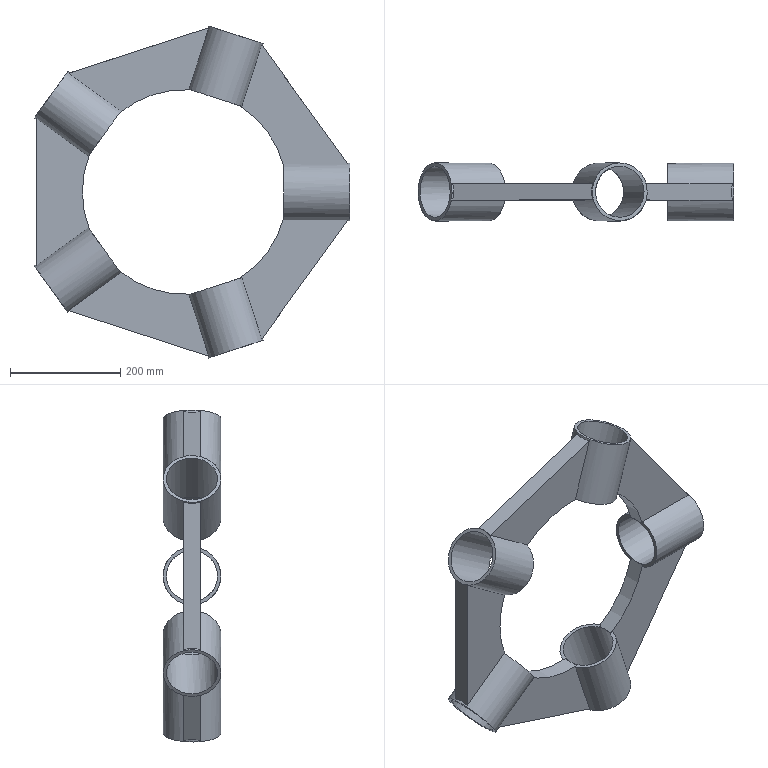Component | NX | RADIAL_ENGINE_PISTON_BLOCK | 1 solid | 45 faces | volume 3767782 mm3 | plane 30 | cylinder 15 | commonest cylinder face diameters 105 x5 93 x5 371.819 x5